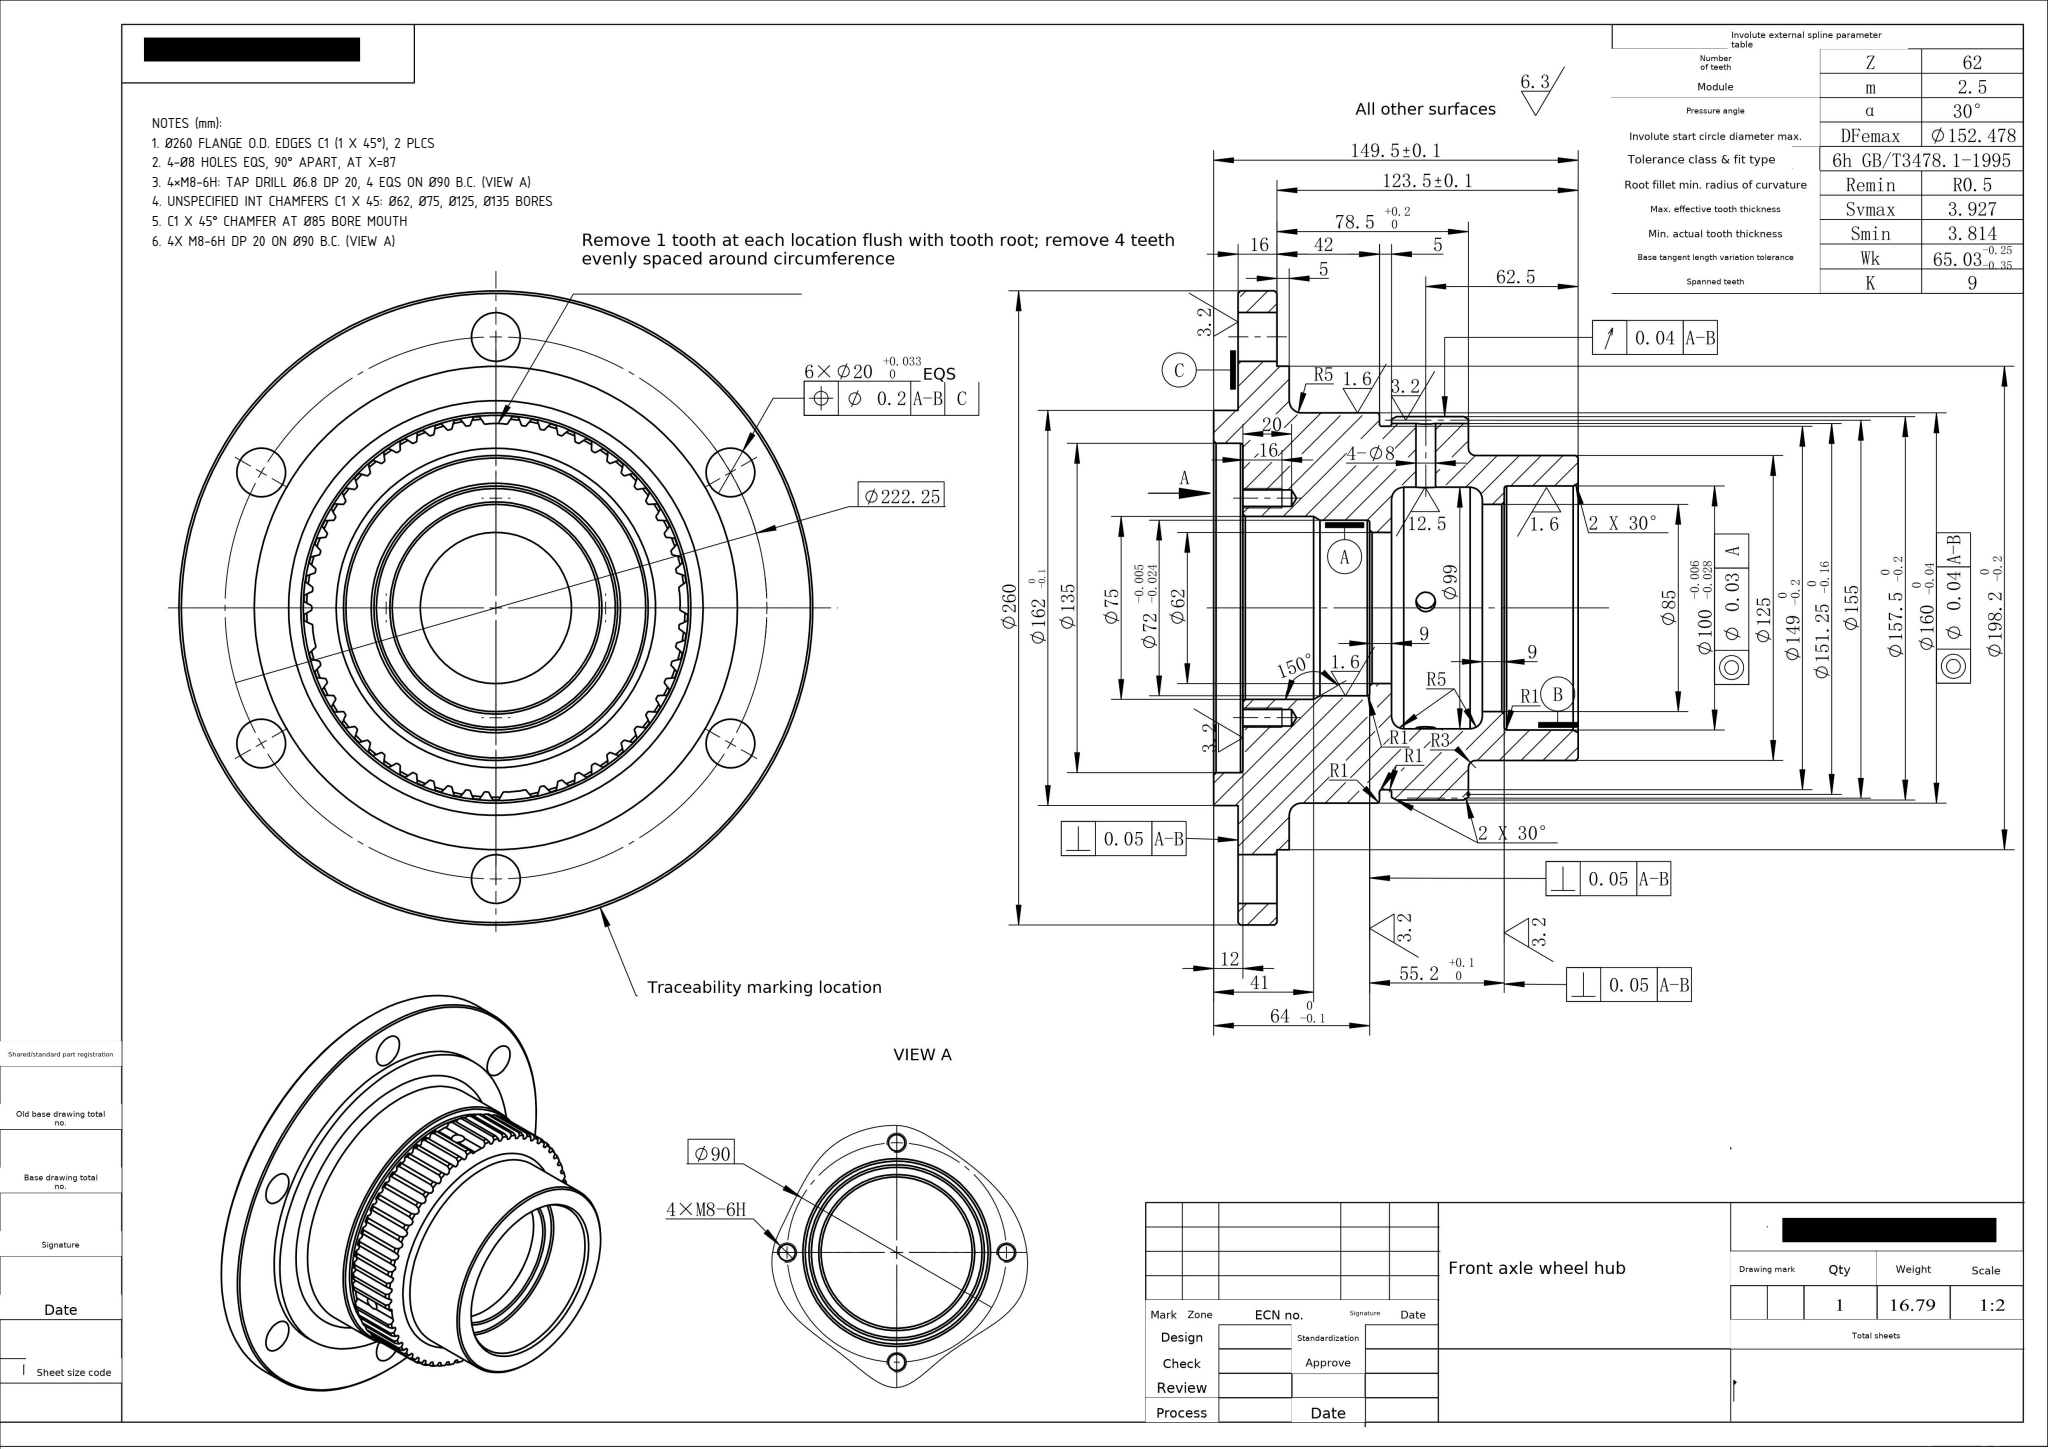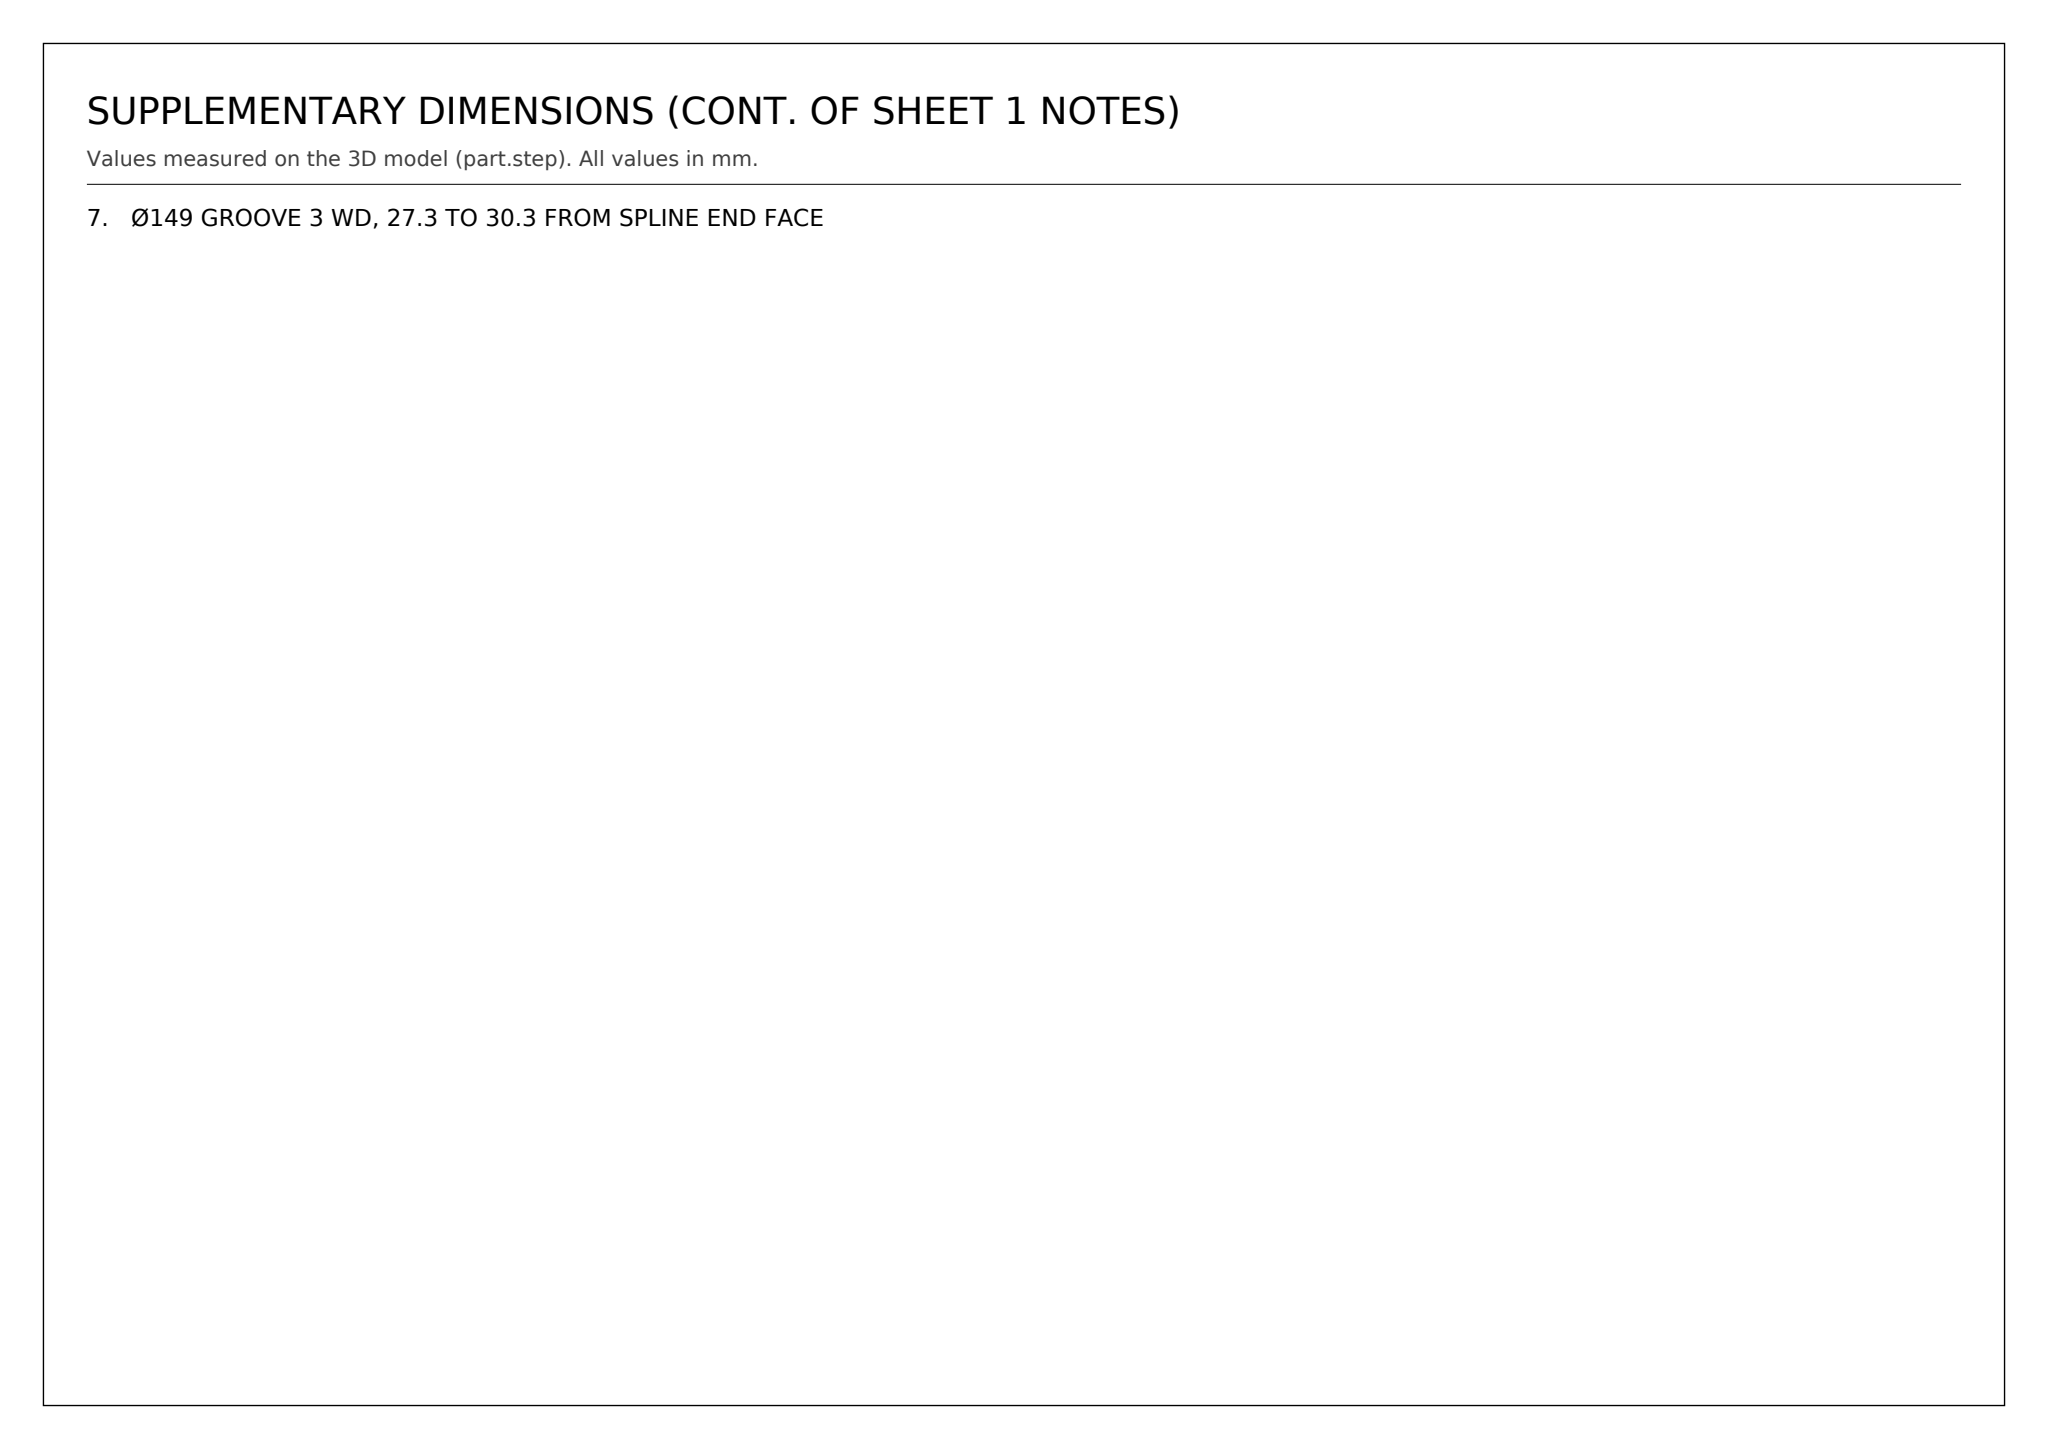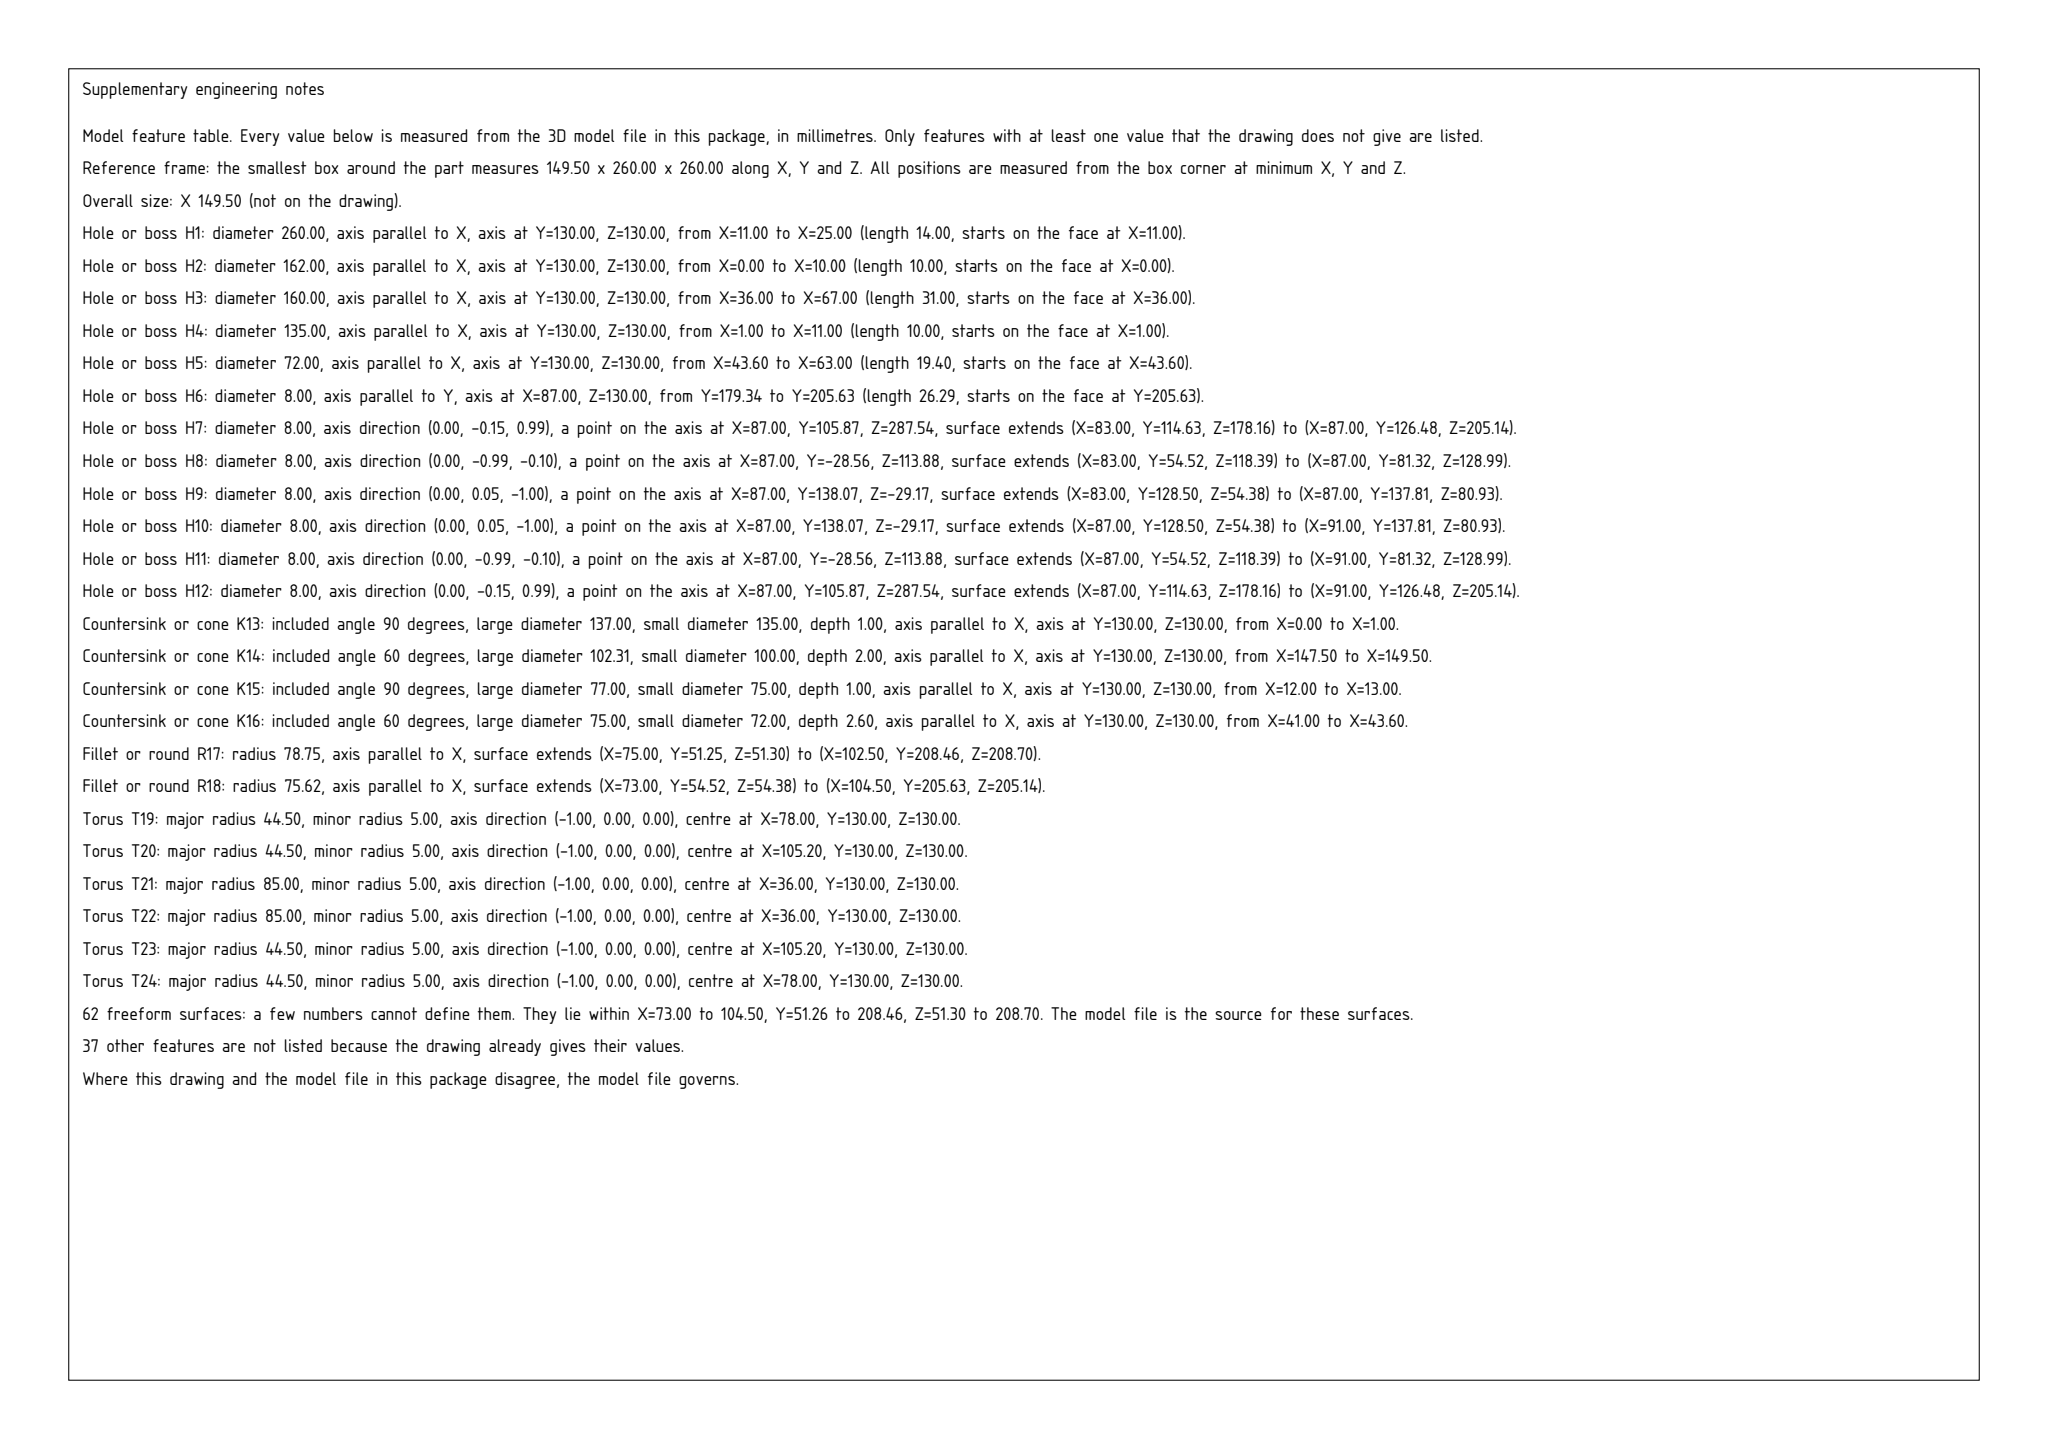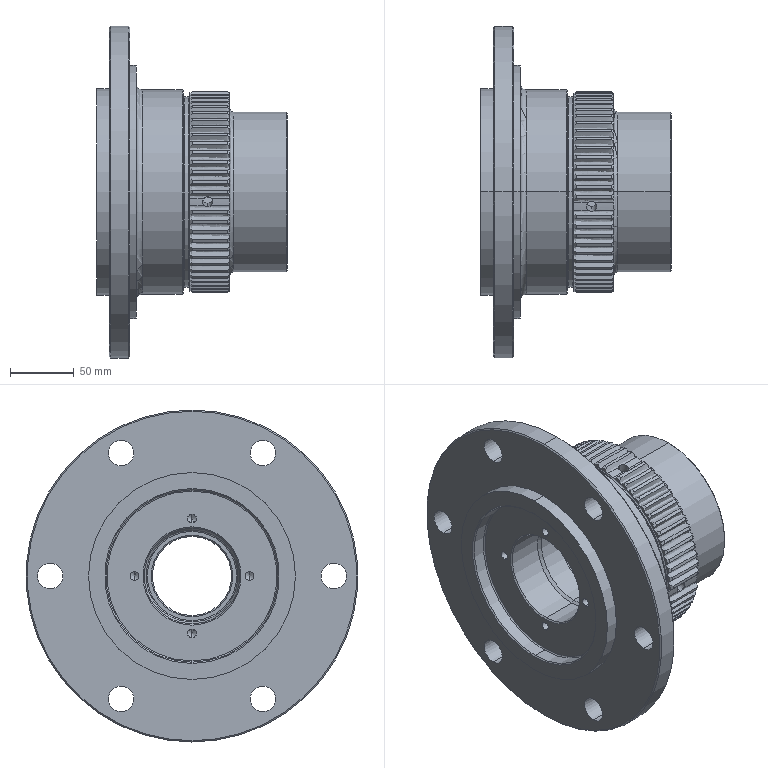Part | SolidWorks | mm | 1 solid | 357 faces | box 149.5 x 260 x 260 mm | volume 2164431 mm3 | cone 142 | cylinder 120 | spline 62 | torus 20 | plane 13 | commonest cylinder face diameters 157.5 x58 20 x12 8 x8 6.8 x8 151.25 x8 135 x2 75 x2 72 x2
Drawing notes:
Ø260 FLANGE O.D. EDGES C1 (1 X 45°), 2 PLCS | from the solid: 90° incl. cones at ref dia 260.0 and 258.0 (x2) on Ø260 flange = 1 mm radial break each side
4-Ø8 HOLES EQS, 90° APART, AT X=87 | from the solid: 4 × Ø8 holes at x=87: 2 axis Y, 2 axis Z (±Y/±Z = 90° spacing)
4×M8-6H: TAP DRILL Ø6.8 DP 20, 4 EQS ON Ø90 B.C. (VIEW A) | from the solid: 4 × Ø6.8 cyl, axis X, len 20.0 w/ 118° drill point at (y,z)=(85,130),(130,85),(130,175),(175,130), R45 from CL (130,130)
UNSPECIFIED INT CHAMFERS C1 X 45: Ø62, Ø75, Ø125, Ø135 BORES | from the solid: cones 90° incl at ref_dia 64 (Ø62 bore), 77 (Ø75 bore), 123 (Ø125 bore), 137 (Ø135 bore) -> 1 mm leg x 45° each
C1 X 45° CHAMFER AT Ø85 BORE MOUTH | from the solid: cones[included_angle,ref_dia] contains [90.0, 85.0] x2 at the Ø85 bore (dia 85, axis x, len 8); 90° incl. = 45° chamfer, 85->87 = C1
4X M8-6H DP 20 ON Ø90 B.C. (VIEW A) | from the solid: 4x Ø6.8 x-axis holes at (85,130),(130,85),(130,175),(175,130) = R45 from axis (130,130) -> Ø90 B.C.; modelled hole depth 20.0 (plus 118° drill point)
Ø149 GROOVE 3 WD, 27.3 TO 30.3 FROM SPLINE END FACE | from the solid: cyl Ø149 axis x, len 3.0; groove wall at x-plane 119.2, spline end face at x=149.5 (bbox 149.5) -> 30.3 and 27.3; Ø157.5 spline cyl len 27.5 runs out at this groove